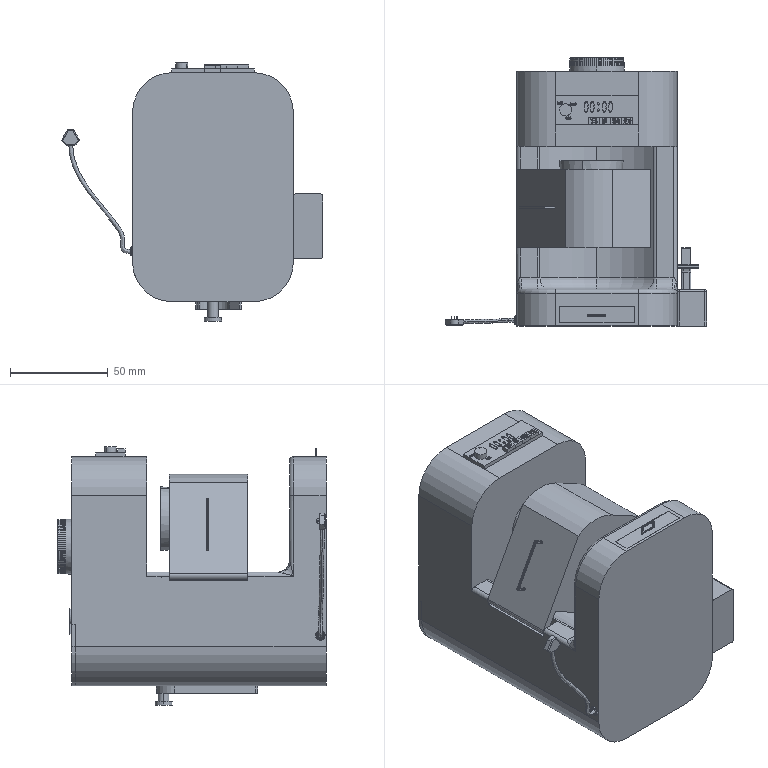Assembly | SolidWorks | mm | 19 component files | 21 solids | 2821 faces | box 133.45 x 137 x 132 mm | volume 734460 mm3 | plane 1716 | spline 529 | cylinder 508 | torus 42 | cone 14 | sphere 12 | commonest cylinder face diameters 0.621 x250 0.4 x37 2 x22 1 x16 1.205 x16 0.2 x14 4 x13 30 x12
Bill of materials:
BeanStorageBox | 1 |  | Flanged bushing-like body: a rounded-square flat flange with a coaxial cylindrical boss on one face and a through bore; a separate smaller tapered ring is shown on the opposite side, offset from the flange.
BeanStorageBoxLid | 1 |  | Thin flat rounded-square plate with a large central circular hole and five small through holes evenly spaced on a circle around it.
BrushHolder | 1 |  | C-shaped (three-sided) bar of rectangular cross-section, with rounded outer corners, filleted inner corners and rounded long edges.
Buckle | 1 |  | Flat ring of constant thickness with one straight rectangular tab sticking out from its outer edge at a slight angle from radial.
Button | 1 |  | Short solid cylinder with flat end faces and a very small raised mark or tab near the edge of one end face.
Button1 | 1 |  | Rectangular block with text characters reading 'NO' as a relief feature on the top face.
Button2 | 1 |  | Rectangular block with text characters reading 'YES' as a relief feature on the top face.
Button3 | 1 |  | Rectangular block with two CJK-style characters as a relief feature on the top face.
Button4 | 1 |  | Rectangular block with two CJK-style characters as a relief feature on the top face.
Clip | 1 |  | Thin flat strip bent into a U/hairpin shape, with a semicircular end and two long, slightly diverging straight legs with open ends.
CoffeeBasketHolder | 1 |  | Housing-like block with a convex curved top surface, a downward lip or leg along one edge, a thin rectangular wire-frame loop on one side, and a small cylindrical pin.
CoffeeCup | 1 |  | Solid tapered cylinder (truncated cone) with flat circular end faces.
GrindingDisc | 1 |  | Stepped cylindrical solid: a smaller-diameter cylinder joined coaxially to a short larger-diameter flange; the smaller end face has many small through-holes or perforations arranged in concentric rings around a plain central area.
MainBody | 1 |  | Rounded-corner block with a deep U-shaped channel cut across it, leaving two upright side walls; one wall has a round through-hole, and there are small pin-like projections, a rectangular pocket on one wall top, and a raised rectangular pad with small character markings on the other wall top.
PowerCord | 1 |  | Long slender flexible-looking cord or rod bent in an S-curve, ending at one end in a flat, roughly pentagonal/shield-shaped head with three small thin pins sticking up from it; the other end is a plain round cut end.
Scoop | 1 |  | T-shaped bar: a long rectangular-section arm with chamfered or rounded edges that blends through large fillets into a wider perpendicular crossbar; thin flat lips or flanges stick out from the crossbar end.
StorageBox | 1 |  | Plain rectangular block (cuboid) with small rounded edges and corners and no other visible features.
WaterStorageBox | 1 |  | Thin, sharp-edged rectangular slab or panel with a small rectangular loop or bail-shaped tab sticking out from the center of one narrow edge.
WaterTankLid | 1 |  | Thin flat plate with one straight long edge and a rounded, D-shaped or half-stadium opposite side; a small rectangular block with two short coaxial cylindrical pins sits on one face near the curved edge.
Mates:
1. concentric | MainBody-1 face at (-76.689, -2.416, 229.26) dir (0, 1, 0) r 23 | BeanStorageBox-2 face at (-76.689, -2.416, 229.26) dir (0, 1, 0) r 23
2. coincident | MainBody-1 face at (-49.714, 12.584, 242.34) dir (-1, 0, 0) | BeanStorageBox-2 face at (-49.714, 12.584, 242.34) dir (1, 0, 0)
3. concentric | MainBody-1 face at (-76.689, 50.251, 229.26) dir (0, -1, 0) r 12.5 | GrindingDisc-1 face at (-76.689, -2.416, 229.26) dir (0, -1, 0) r 12.5
4. coincident | MainBody-1 face at (-76.689, -2.416, 229.26) dir (0, 1, 0) | GrindingDisc-1 face at (-76.689, -2.416, 229.26) dir (0, -1, 0)
5. coincident | MainBody-1 face at (-76.689, -2.416, 229.26) dir (0, 1, 0) | BeanStorageBox-2 face at (-76.689, -2.416, 229.26) dir (0, -1, 0)
6. concentric | BeanStorageBox-2 face at (-76.689, 14.584, 229.26) dir (0, 1, 0) r 52.36 | BeanStorageBoxLid-1 face at (-76.689, 20.584, 229.26) dir (0, 1, 0) r 14.25
7. concentric | MainBody-1 face at (-64.714, 12.584, 242.34) dir (0, 1, 0) r 15 | BeanStorageBoxLid-1 face at (-64.714, 22.584, 242.34) dir (0, -1, 0) r 15
8. concentric | MainBody-1 face at (-68.689, 18.584, 159.753) dir (-1, 0, 0) r 0.9 | WaterTankLid-2 face at (-68.689, 18.584, 159.753) dir (-1, 0, 0) r 0.9
9. coincident | MainBody-1 face at (-68.689, 18.584, 159.753) dir (-1, 0, 0) | WaterTankLid-2 face at (-68.689, 18.584, 159.753) dir (1, 0, 0)
10. concentric | MainBody-1 face at (-115.859, -23.396, 213.782) dir (0, -1, 0) r 1.375 | CoffeeBasketHolder-1 face at (-115.859, -23.396, 213.782) dir (0, -1, 0) r 1.375
11. coincident | MainBody-1 face at (-115.859, -23.396, 213.782) dir (0, -1, 0) | CoffeeBasketHolder-1 face at (-115.859, -23.396, 213.782) dir (0, 1, 0)
12. coincident | CoffeeCup-1 face at (-66.675, -65.396, 247.378) dir (0, -1, 0) | CoffeeBasketHolder-1 face at (-61.856, -65.396, 263.104) dir (0, 1, 0)
13. concentric | CoffeeCup-1 edge at (-79.558, -23.012, 243.54) dir (0, -1, 0) r 16.271 | CoffeeBasketHolder-1 edge at (-79.558, -27.396, 243.54) dir (0, -1, 0) r 18.617
14. coincident | BeanStorageBox-2 face at (-88.664, 20.584, 216.18) dir (0, 1, 0) | BeanStorageBoxLid-1 face at (-64.714, 20.584, 216.18) dir (0, -1, 0)
15. coincident | MainBody-1 face at (-55.654, 20.584, 178.253) dir (0, 1, 0) | WaterTankLid-2 face at (-76.707, 20.584, 216.702) dir (0, -1, 0)
16. concentric | MainBody-1 face at (-112.724, -104.464, 183.909) dir (-1, 0, 0) r 1 | PowerCord-3 face at (-112.724, -104.464, 183.909) dir (-1, 0, 0) r 1
17. coincident | MainBody-1 face at (-112.724, -104.464, 183.909) dir (-1, 0, 0) | PowerCord-3 face at (-112.724, -104.464, 183.909) dir (1, 0, 0)
18. coincident | MainBody-1 face at (-97.724, -107.416, 255.152) dir (0, -1, 0) | StorageBox-1 face at (-20.654, -107.416, 213.244) dir (0, -1, 0)
19. coincident | MainBody-1 face at (-35.654, 22.584, 255.152) dir (1, 0, 0) | StorageBox-1 face at (-35.654, -107.416, 213.244) dir (-1, 0, 0)
20. distance | StorageBox-1 face at (-20.654, -107.416, 213.244) dir (0, 0, 1) | MainBody-1 face at (-165.654, -15.749, 216.244) dir (0, 0, 1)
21. coincident | MainBody-1 face at (-95.786, -97.312, 221.152) dir (1, 0, 0) | WaterStorageBox-1 face at (-95.786, -105.84, 275.205) dir (-1, 0, 0)
22. coincident | MainBody-1 edge at (-95.786, -105.84, 275.152) dir (1, 0, 0) | WaterStorageBox-1 face at (-95.786, -105.84, 275.205) dir (0, -1, 0)
23. coincident | MainBody-1 face at (-95.786, -105.84, 221.152) dir (0, 1, 0) | WaterStorageBox-1 edge at (-95.786, -105.84, 221.205) dir (1, 0, 0)
24. distance | StorageBox-1 face at (-20.654, -107.416, 213.244) dir (0, 0, 1) | BrushHolder-1 face at (-35.654, -78.145, 207.244) dir (0, 0, 1)
25. distance | BrushHolder-1 face at (-35.654, -78.145, 205.244) dir (0, -1, 0) | StorageBox-1 face at (-20.654, -88.687, 213.244) dir (0, 1, 0)
26. coincident | BrushHolder-1 face at (-35.654, -76.145, 205.244) dir (0, 1, 0) | Scoop-1 face at (-28.654, -76.145, 209.929) dir (0, -1, 0)
27. concentric | MainBody-1 face at (-92.68, 2.928, 279.152) dir (0, 0, -1) r 0.5 | Button-1 face at (-92.68, 2.928, 279.152) dir (0, 0, -1) r 0.5
28. coincident | MainBody-1 face at (-92.68, 2.928, 279.152) dir (0, 0, 1) | Button-1 face at (-92.68, 2.928, 279.152) dir (0, 0, -1)
29. coincident | MainBody-1 face at (-97.724, 22.584, 158.253) dir (0, 0, -1) | Clip-1 face at (-76.241, -30.023, 158.253) dir (0, 0, 1)
30. coincident | StorageBox-1 face at (-33.654, -106.687, 182.244) dir (1, 0, 0) | Scoop-1 face at (-33.654, -80.145, 190.299) dir (-1, 0, 0)
31. distance | Scoop-1 face at (-28.654, -76.145, 209.929) dir (0, 0, 1) | BrushHolder-1 face at (-35.654, -78.145, 207.244) dir (0, 0, 1)
32. coincident | MainBody-1 face at (-35.654, 22.584, 255.152) dir (1, 0, 0) | BrushHolder-1 face at (-35.654, -78.145, 205.244) dir (-1, 0, 0)
33. coincident | MainBody-1 face at (-76.689, -107.416, 277.152) dir (0, 0, 1) | Button1-1 face at (-75.506, -4.714, 277.152) dir (0, 0, -1)
34. coincident | MainBody-1 face at (-76.689, -107.416, 277.152) dir (0, 0, 1) | Button4-1 face at (-69.806, -4.714, 277.152) dir (0, 0, -1)
35. coincident | MainBody-1 face at (-76.689, -107.416, 277.152) dir (0, 0, 1) | Button2-1 face at (-81.206, -4.714, 277.152) dir (0, 0, -1)
36. coincident | MainBody-1 face at (-76.689, -107.416, 277.152) dir (0, 0, 1) | Button3-1 face at (-64.106, -4.714, 277.152) dir (0, 0, -1)
37. coincident | MainBody-1 face at (-97.724, -4.714, 277.152) dir (0, -1, 0) | Button1-1 face at (-75.506, -4.714, 279.152) dir (0, -1, 0)
38. coincident | MainBody-1 face at (-97.724, -4.714, 277.152) dir (0, -1, 0) | Button3-1 face at (-64.106, -4.714, 279.152) dir (0, -1, 0)
39. coincident | MainBody-1 face at (-97.724, -4.714, 277.152) dir (0, -1, 0) | Button4-1 face at (-69.806, -4.714, 279.152) dir (0, -1, 0)
40. coincident | MainBody-1 face at (-97.724, -4.714, 277.152) dir (0, -1, 0) | Button2-1 face at (-81.206, -4.714, 279.152) dir (0, -1, 0)
41. coincident | Button1-1 edge at (-75.506, -1.014, 279.152) dir (0, -1, 0) | Button2-1 edge at (-75.506, -4.714, 279.152) dir (0, 1, 0)
42. coincident | Button1-1 face at (-75.506, -4.714, 279.152) dir (0, 0, 1) | Button4-1 edge at (-69.806, -1.014, 279.152) dir (0, -1, 0)
43. coincident | Button3-1 edge at (-64.106, -1.014, 279.152) dir (0, -1, 0) | Button4-1 edge at (-64.106, -4.714, 279.152) dir (0, 1, 0)
44. concentric | MainBody-1 face at (-76.689, 23.584, 193.489) dir (0, -1, 0) r 2.5 | Buckle-1 face at (-76.689, 23.584, 193.489) dir (0, -1, 0) r 2.5
45. coincident | MainBody-1 face at (-97.724, 22.584, 255.152) dir (0, 1, 0) | Buckle-1 face at (-76.689, 22.584, 193.489) dir (0, -1, 0)
46. coincident | Button1-1 face at (-69.806, -4.714, 279.152) dir (1, 0, 0) | Button4-1 face at (-69.806, -4.714, 279.152) dir (-1, 0, 0)